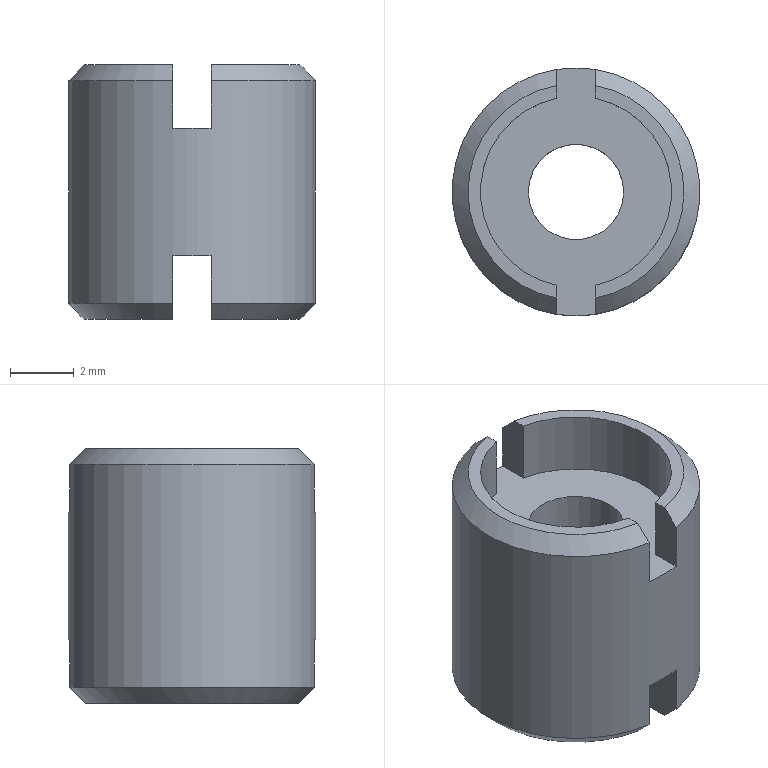Component | NX | DXF_04_ADJUSTING_SCREW | 1 solid | 23 faces | volume 261 mm3 | plane 15 | cylinder 4 | cone 4 | commonest cylinder face diameters 6 x2 7.785 x1 3 x1